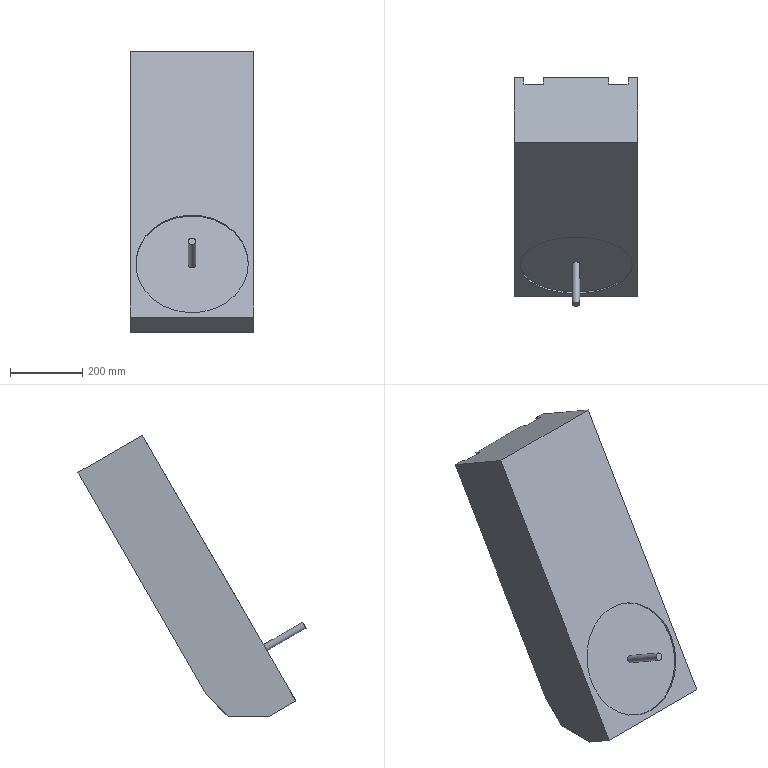Component | NX | SIM15_X1_SCHLITTEN | 1 solid | 20 faces | volume 56433503 mm3 | plane 18 | cylinder 2 | commonest cylinder face diameters 312 x1 20 x1